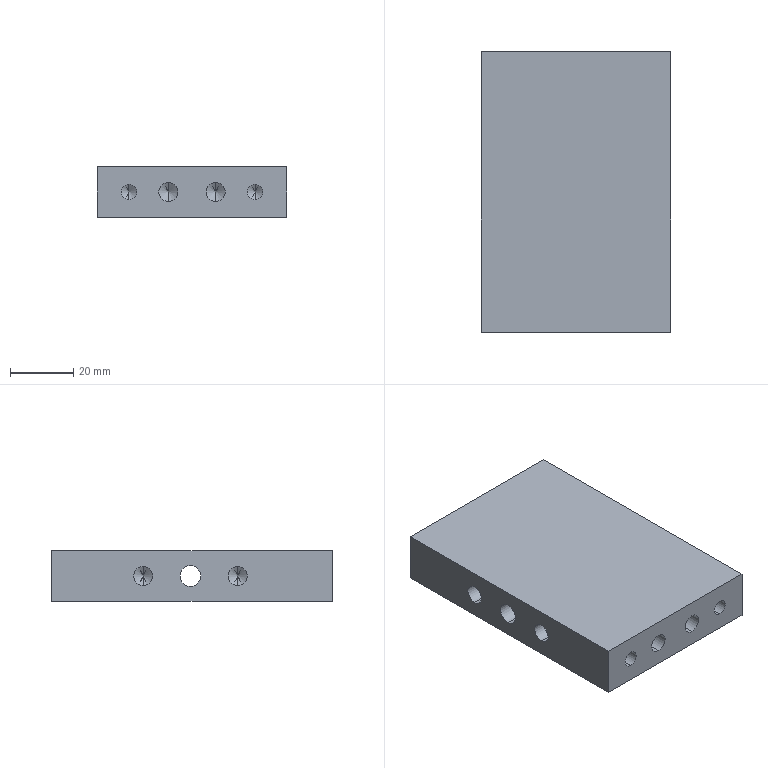Component | SolidWorks | UnitFixingSeat2-002-1 | 1 solid | 43 faces | box 60 x 89 x 16 mm | volume 76328 mm3 | cylinder 20 | cone 16 | plane 7 | commonest cylinder face diameters 5 x8 6 x8 11 x2 6.6 x2 | material 6061 Alloy
build123d program:
from build123d import *

# Parameters (mm, degrees)
SKETCH2_W                                          = 60
SKETCH2_H                                          = 89
BOSS_EXTRUDE1_DEPTH                                = 8
F_6_0_6_DIAMETER_HOLE1_D                           = 6
F_6_0_6_DIAMETER_HOLE1_DEPTH                       = 20
F_6_0_6_DIAMETER_HOLE1_TIP                         = 1.803
F_6_0_6_DIAMETER_HOLE2_D                           = 6
F_6_0_6_DIAMETER_HOLE2_DEPTH                       = 20
F_6_0_6_DIAMETER_HOLE2_TIP                         = 1.803
M6_TAPPED_HOLE2_D                                  = 5
M6_TAPPED_HOLE2_DEPTH                              = 21
M6_TAPPED_HOLE2_TIP                                = 1.502
M6_TAPPED_HOLE3_D                                  = 5
M6_TAPPED_HOLE3_DEPTH                              = 21
M6_TAPPED_HOLE3_TIP                                = 1.502
HOLE_SIZE_ACCORDING_TO_TYPE_0_OF_HEXAG_D           = 6.6
HOLE_SIZE_ACCORDING_TO_TYPE_0_OF_HEXAG_CBORE_D     = 11
HOLE_SIZE_ACCORDING_TO_TYPE_0_OF_HEXAG_CBORE_DEPTH = 50


with BuildPart() as part:
    # Sketch2 → Boss-Extrude1 (new, symmetric)
    with BuildSketch(Plane.XY):
        Rectangle(SKETCH2_W, SKETCH2_H)
    extrude(amount=BOSS_EXTRUDE1_DEPTH, both=True)

    # 6.0 _6_ Diameter Hole1
    with Locations(Plane.ZY.offset(30)):
        with Locations((0, -14.5), (0, 15.5)):
            Hole(F_6_0_6_DIAMETER_HOLE1_D / 2, depth=F_6_0_6_DIAMETER_HOLE1_DEPTH)
            with Locations((0, 0, -(F_6_0_6_DIAMETER_HOLE1_DEPTH + F_6_0_6_DIAMETER_HOLE1_TIP / 2))):  # 118° drill point
                Cone(0, F_6_0_6_DIAMETER_HOLE1_D / 2, F_6_0_6_DIAMETER_HOLE1_TIP, mode=Mode.SUBTRACT)

    # 6.0 _6_ Diameter Hole2
    with Locations(Plane(origin=(0, -44.5, 0), x_dir=(-1, 0, 0), z_dir=(0, -1, 0))):
        with Locations((-7.5, 0), (7.5, 0)):
            Hole(F_6_0_6_DIAMETER_HOLE2_D / 2, depth=F_6_0_6_DIAMETER_HOLE2_DEPTH)
            with Locations((0, 0, -(F_6_0_6_DIAMETER_HOLE2_DEPTH + F_6_0_6_DIAMETER_HOLE2_TIP / 2))):  # 118° drill point
                Cone(0, F_6_0_6_DIAMETER_HOLE2_D / 2, F_6_0_6_DIAMETER_HOLE2_TIP, mode=Mode.SUBTRACT)

    # M6 Tapped Hole2
    with Locations(Plane(origin=(0, -44.5, 0), x_dir=(-1, 0, 0), z_dir=(0, -1, 0))):
        with Locations((-20, 0), (20, 0)):
            Hole(M6_TAPPED_HOLE2_D / 2, depth=M6_TAPPED_HOLE2_DEPTH)
            with Locations((0, 0, -(M6_TAPPED_HOLE2_DEPTH + M6_TAPPED_HOLE2_TIP / 2))):  # 118° drill point
                Cone(0, M6_TAPPED_HOLE2_D / 2, M6_TAPPED_HOLE2_TIP, mode=Mode.SUBTRACT)

    # M6 Tapped Hole3
    with Locations(Plane(origin=(0, 44.5, 0), x_dir=(1, 0, 0), z_dir=(0, 1, 0))):
        with Locations((-10, 0), (20, 0)):
            Hole(M6_TAPPED_HOLE3_D / 2, depth=M6_TAPPED_HOLE3_DEPTH)
            with Locations((0, 0, -(M6_TAPPED_HOLE3_DEPTH + M6_TAPPED_HOLE3_TIP / 2))):  # 118° drill point
                Cone(0, M6_TAPPED_HOLE3_D / 2, M6_TAPPED_HOLE3_TIP, mode=Mode.SUBTRACT)

    # Hole Size _according to_ Type 0 of Hexag (through all)
    with Locations(Plane(origin=(30, 0, 0), x_dir=(0, 0, -1), z_dir=(1, 0, 0))):
        with Locations((0, 0.5)):
            CounterBoreHole(HOLE_SIZE_ACCORDING_TO_TYPE_0_OF_HEXAG_D / 2, HOLE_SIZE_ACCORDING_TO_TYPE_0_OF_HEXAG_CBORE_D / 2, HOLE_SIZE_ACCORDING_TO_TYPE_0_OF_HEXAG_CBORE_DEPTH)


solid = part.part

# Placed as in the assembly
solid = solid.moved(Location((31.028, -16.399, 117.932), (0, 0, 0)))